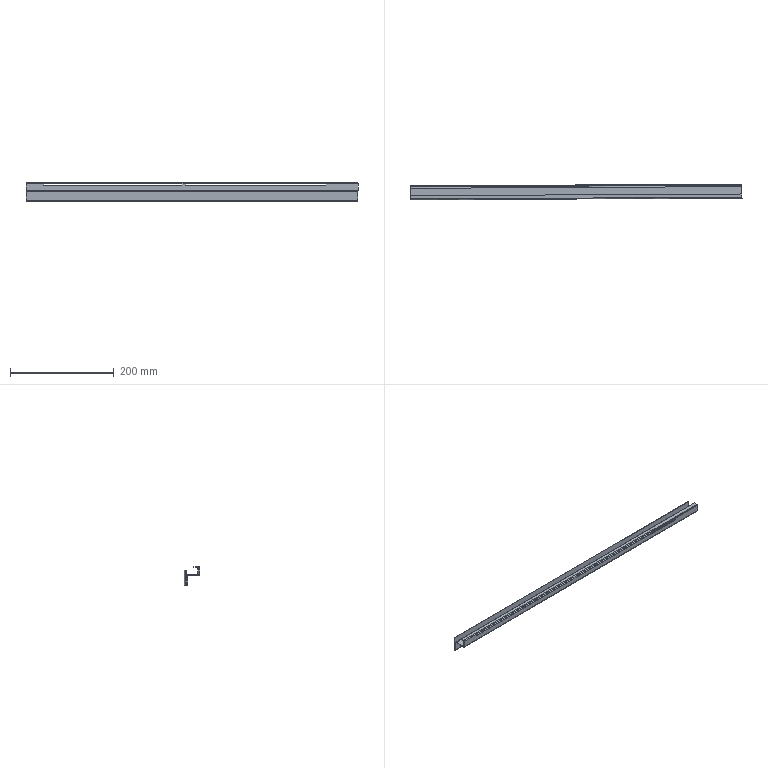Component | SolidWorks | RAY MONTAJ-1_RAY SOL-2 | 1 solid | 55 faces | volume 57422 mm3 | plane 45 | cylinder 10 | commonest cylinder face diameters 1.473 x5 3.473 x5